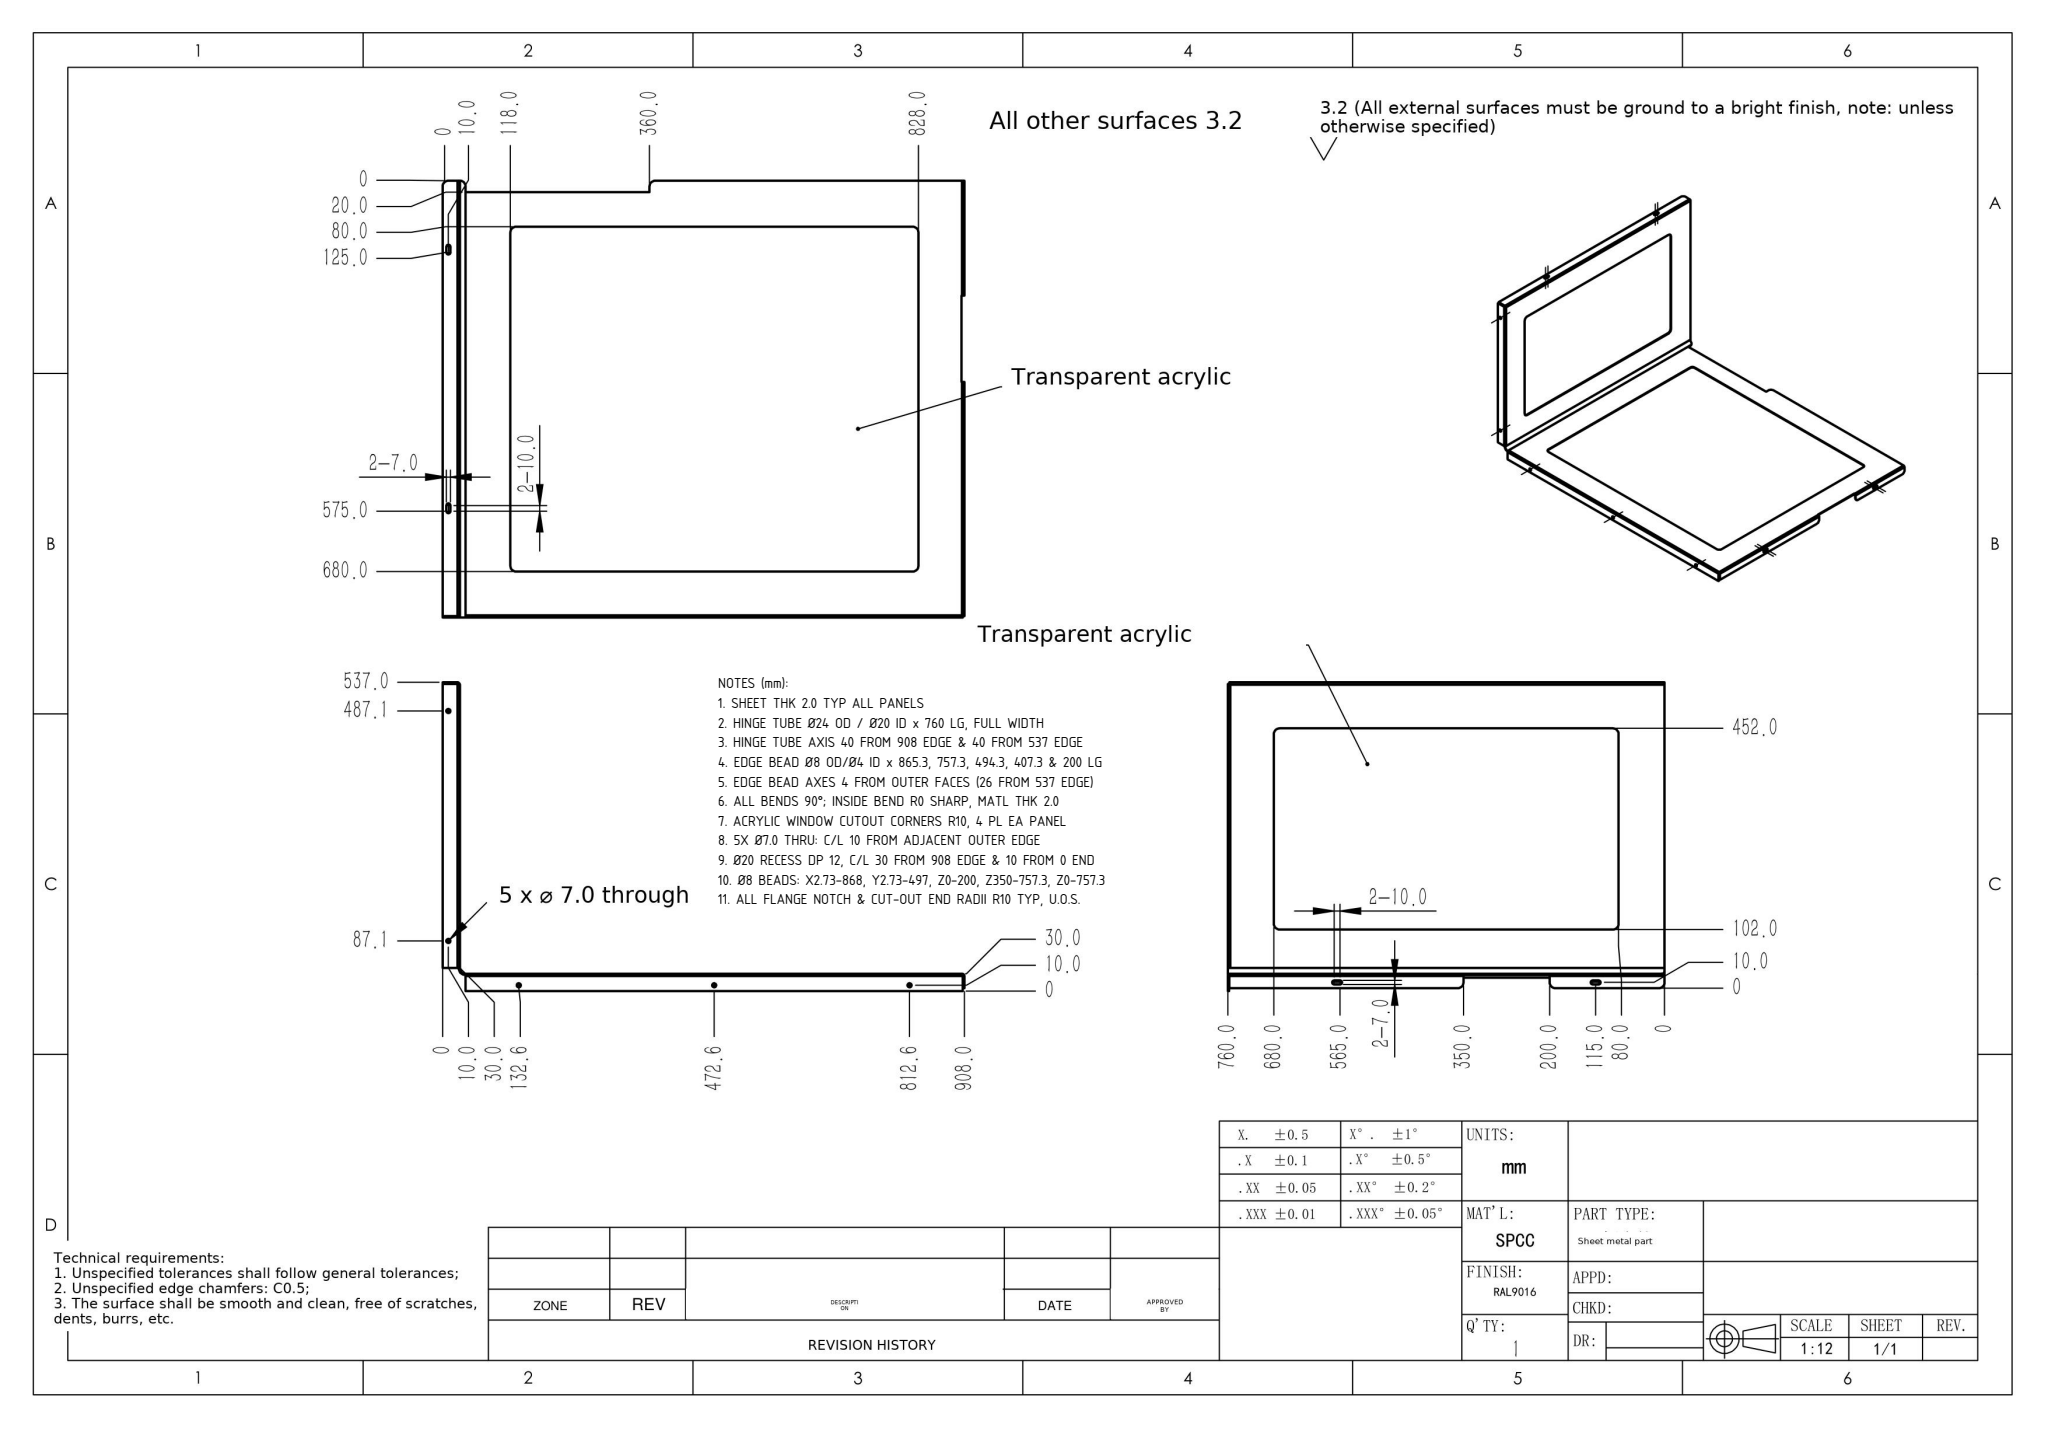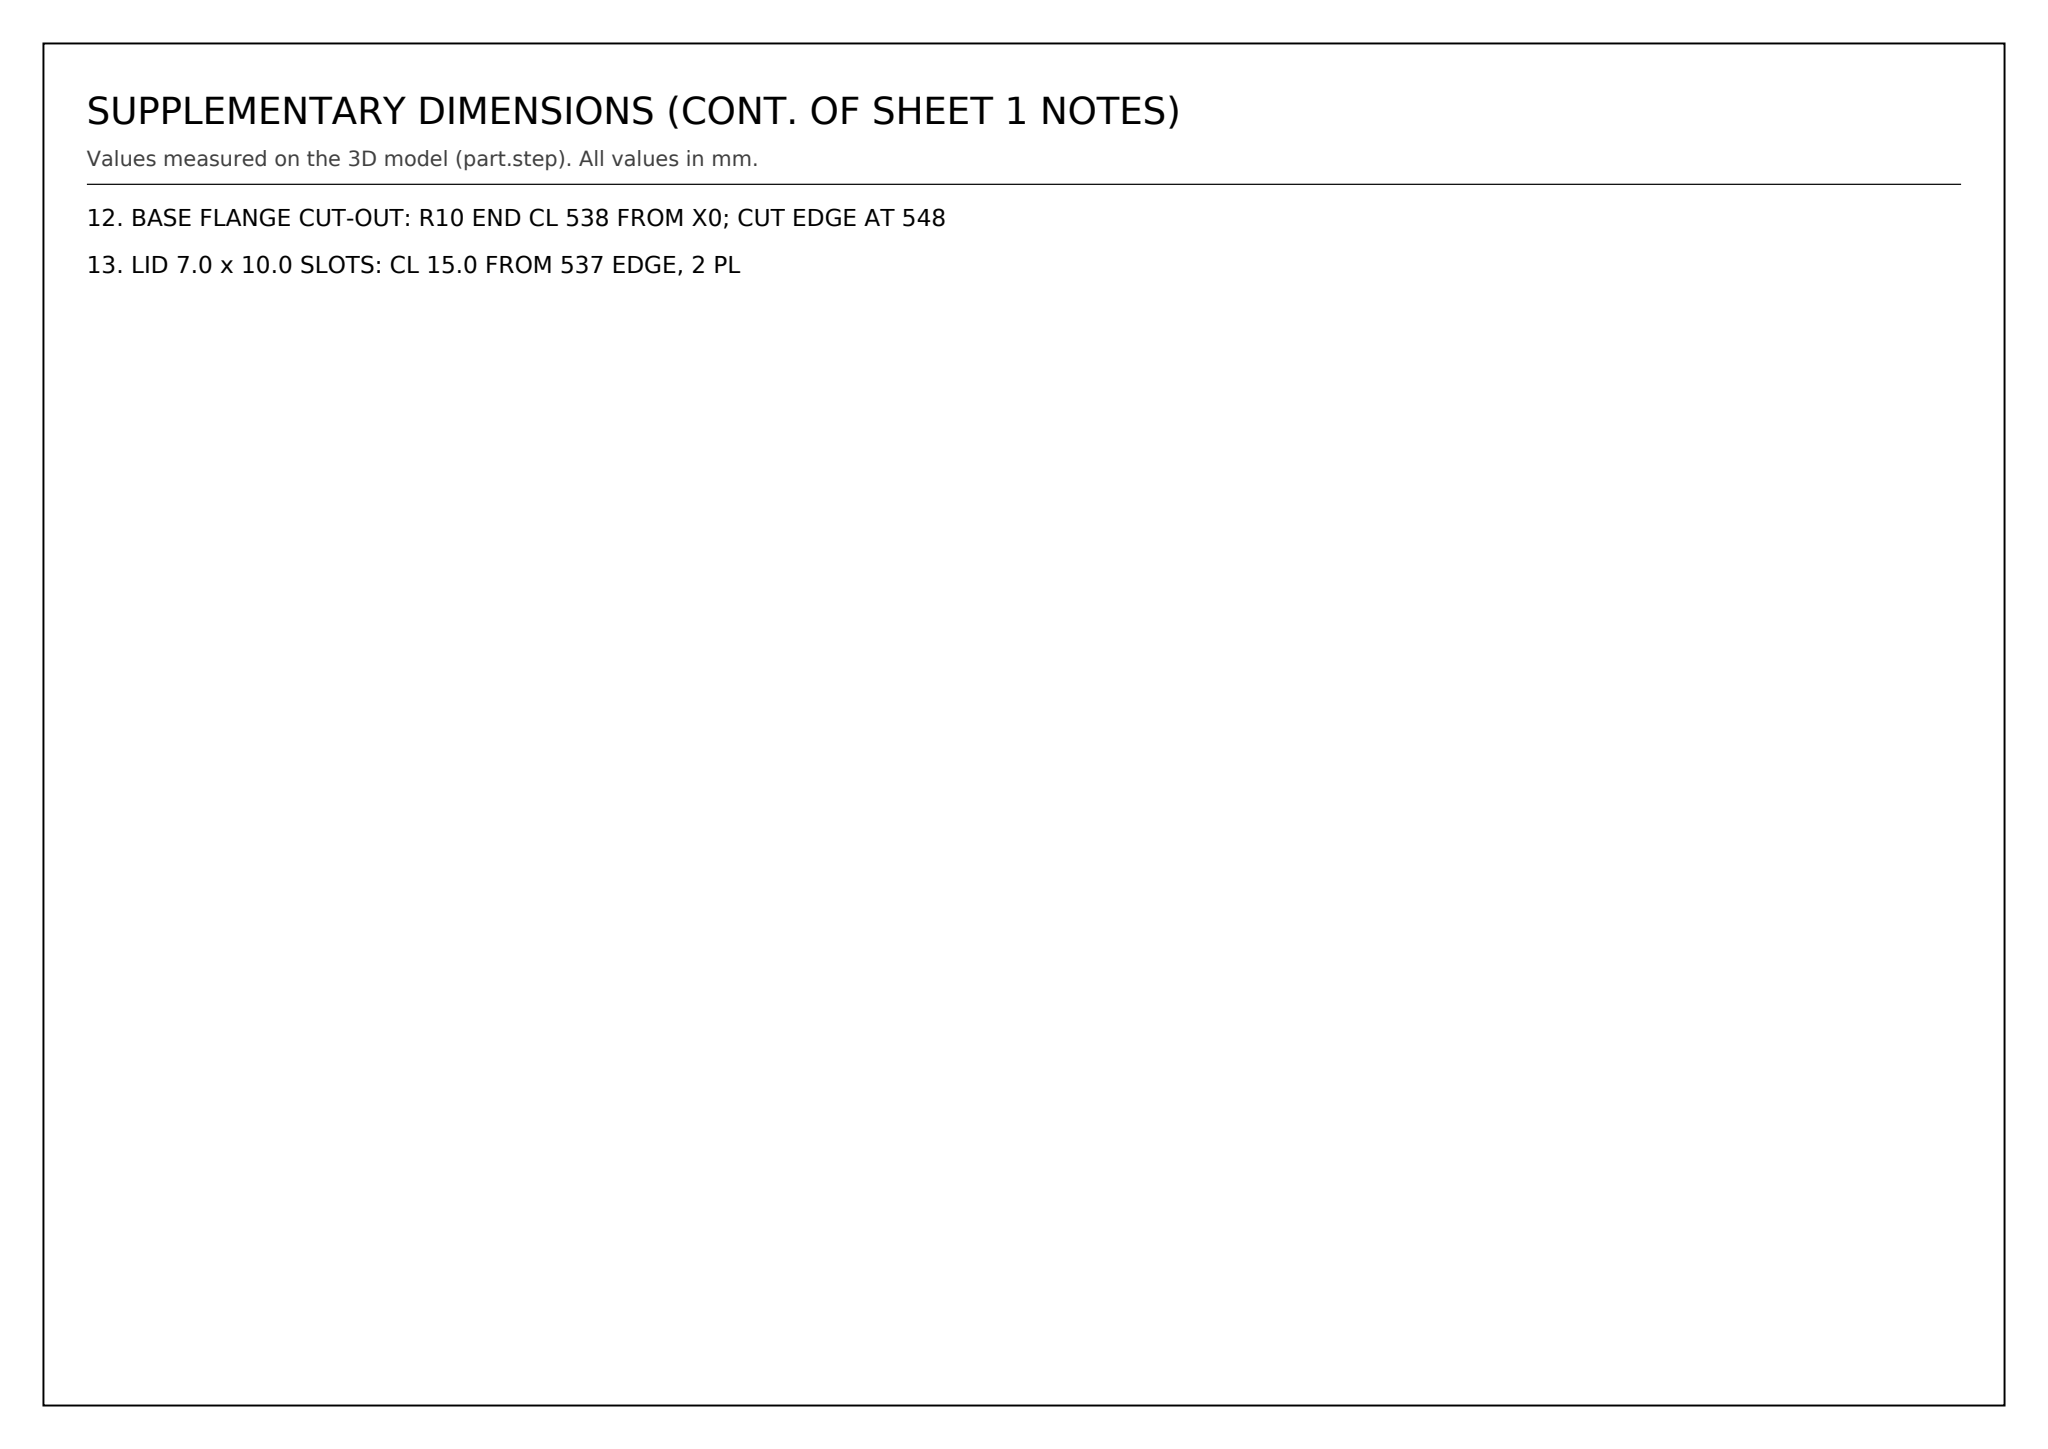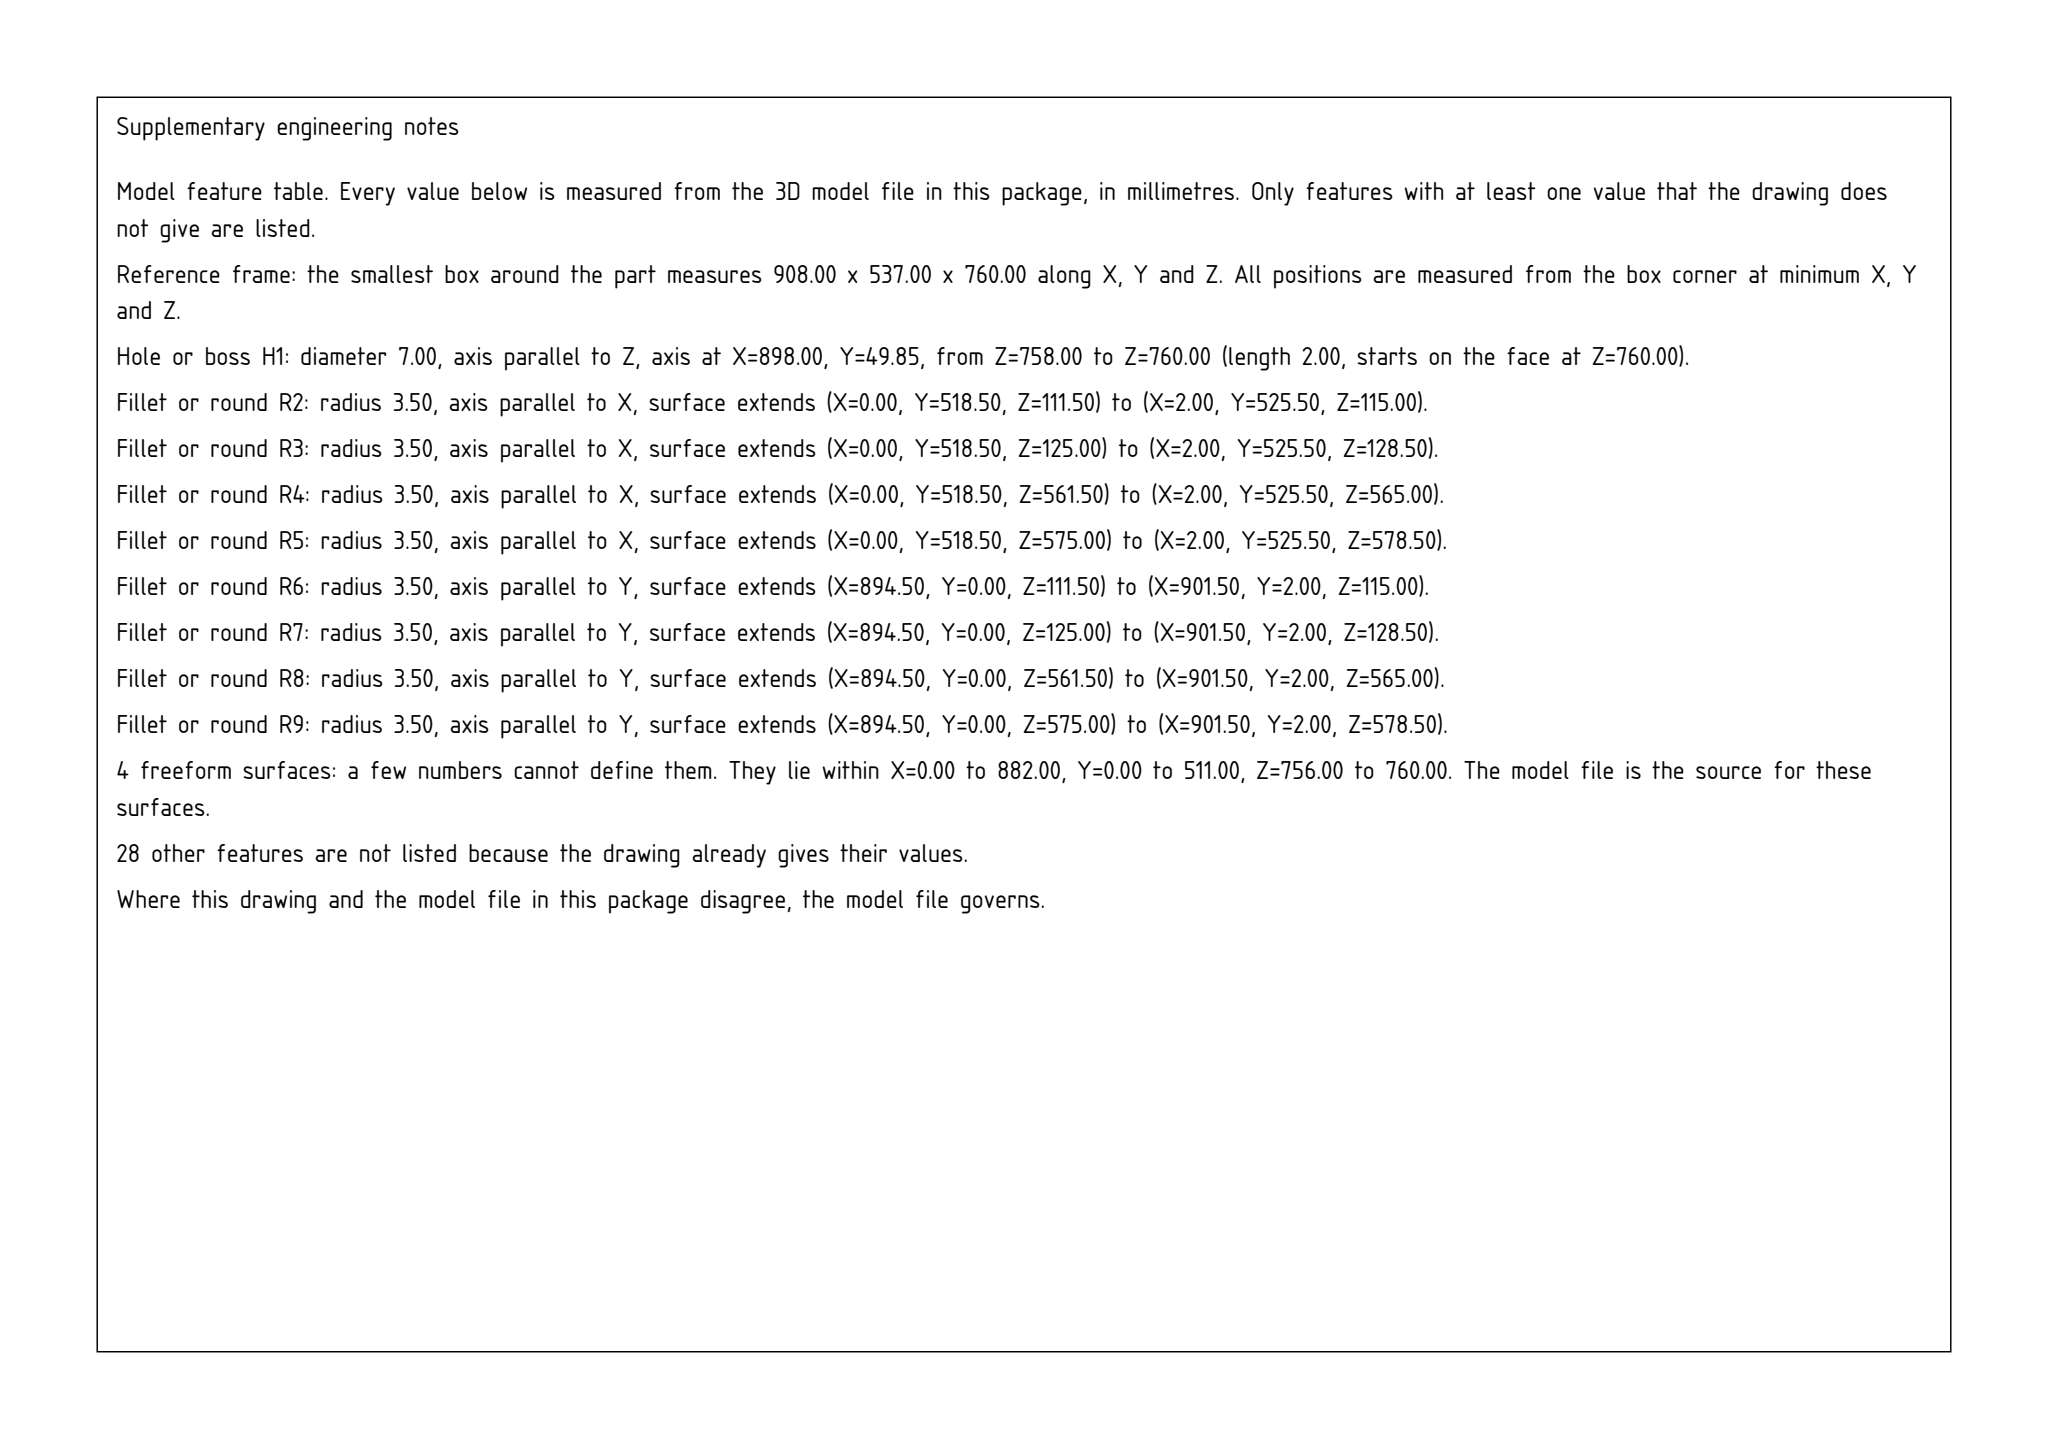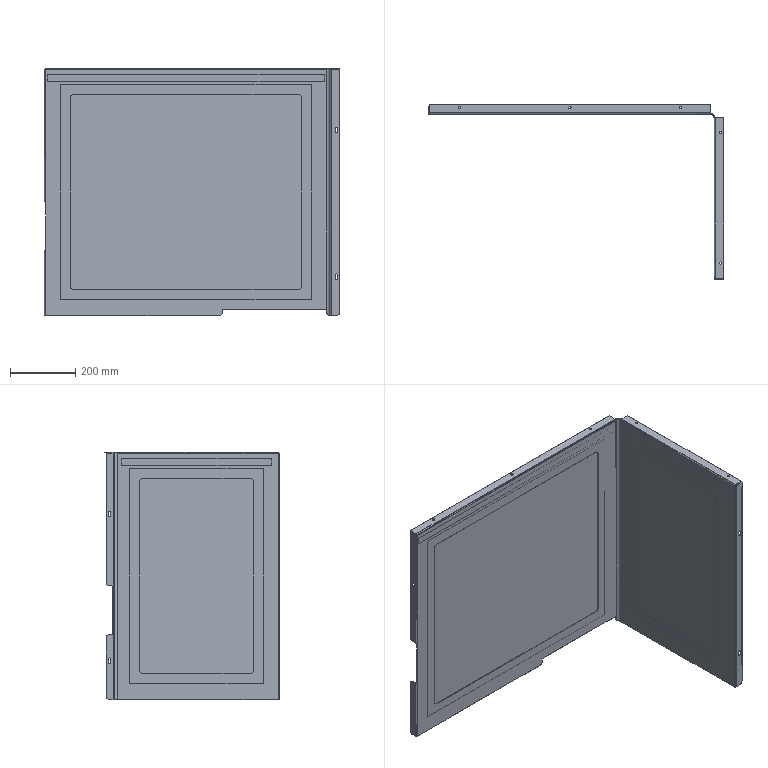Part | SolidWorks | mm | 1 solid | 129 faces | box 908 x 537 x 760 mm | volume 5109013 mm3 | plane 81 | cylinder 44 | spline 4 | commonest cylinder face diameters 7 x18 20 x15 8 x5 4 x5 24 x1
Drawing notes:
SHEET THK 2.0 TYP ALL PANELS | from the solid: Parallel face pairs x=0.02/2.02, y=0.02/2.02; all Ø7 holes 2.0 deep
HINGE TUBE Ø24 OD / Ø20 ID x 760 LG, FULL WIDTH | from the solid: cyl 24 & 20, axis z, pos (868.02,497.02), length 760
HINGE TUBE AXIS 40 FROM 908 EDGE & 40 FROM 537 EDGE | from the solid: axis x=868.02 (908.02-40), y=497.02 (537.02-40)
EDGE BEAD Ø8 OD/Ø4 ID x 865.3, 757.3, 494.3, 407.3 & 200 LG | from the solid: cyl 8/4 pairs: lengths 865.29, 757.29, 494.29, 407.29, 200.0
EDGE BEAD AXES 4 FROM OUTER FACES (26 FROM 537 EDGE) | from the solid: bead axes at x=4.02/882.02, y=4.02/511.02, z=756 vs bbox 908.02/537.02/760.02
ALL BENDS 90°; INSIDE BEND R0 SHARP, MATL THK 2.0 | from the solid: fillet_radii empty; orthogonal plane sets x/y/z, thk 2.0
ACRYLIC WINDOW CUTOUT CORNERS R10, 4 PL EA PANEL | from the solid: Ø20 x 2.0 cyls at (y=90.02/420.02, z=90/670) and (x=90.02/780.02, z=90/670)
5X Ø7.0 THRU: C/L 10 FROM ADJACENT OUTER EDGE | from the solid: Ø7 z-axis holes at y=527.02 (537.02-10) and x=898.02 (908.02-10)
Ø20 RECESS DP 12, C/L 30 FROM 908 EDGE & 10 FROM 0 END | from the solid: cyl 20, axis y, pos (878.02, z=10), length 12.0
Ø8 BEADS: X2.73-868, Y2.73-497, Z0-200, Z350-757.3, Z0-757.3 | from the solid: Ø8/Ø4 cyl: x-axis L865.29 (2.73->868.02) @y511,z756; y-axis L494.29 (2.73->497.02) @x882,z756; z-axis @x4,y511 L200 (0->200) & L407.29 (350->757.29); z-axis @x882,y4 L757.29 (0->757.29)
ALL FLANGE NOTCH & CUT-OUT END RADII R10 TYP, U.O.S. | from the solid: Ø20 x 2.0 long cylinders at all notch/cut-out ends (e.g. x-axis @y522 z10/190/360; y-axis @x90/780 z90/670) = R10
BASE FLANGE CUT-OUT: R10 END CL 538 FROM X0; CUT EDGE AT 548 | from the solid: Ø20 y-axis cyl at x=538.02, z=10.0, L2.0; plane x=548.02 (bbox min x = 0 datum)
LID 7.0 x 10.0 SLOTS: CL 15.0 FROM 537 EDGE, 2 PL | from the solid: Ø7 x-axis holes at y=522.02, z=115/125 & 565/575; 537.02-522.02 = 15.0 from 537 edge